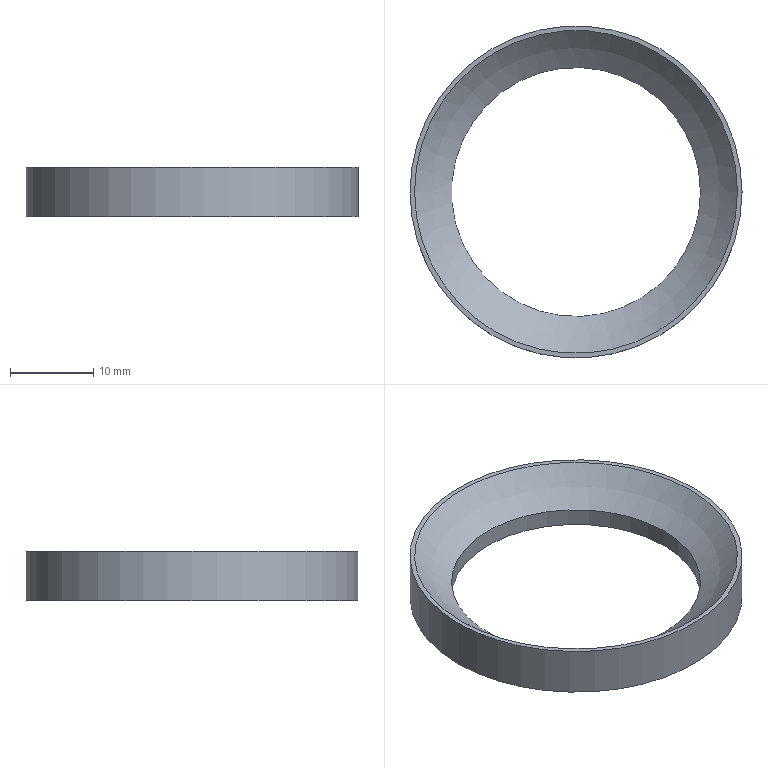Component | NX | CORE_SEAL_2 | 1 solid | 5 faces | box 40 x 40 x 6 mm | volume 2343 mm3 | plane 2 | cylinder 2 | sphere 1 | commonest cylinder face diameters 40 x1 30 x1
STEP:
#1=CARTESIAN_POINT('',(0.,0.,0.));
#2=DIRECTION('',(0.,0.,1.));
#3=DIRECTION('',(1.,0.,0.));
#4=AXIS2_PLACEMENT_3D('',#1,#2,#3);
#5=CARTESIAN_POINT('',(19.449,0.,-45.));
#6=VERTEX_POINT('',#5);
#7=CARTESIAN_POINT('',(0.,0.,-45.));
#8=DIRECTION('',(0.,0.,1.));
#9=DIRECTION('',(1.,0.,0.));
#10=AXIS2_PLACEMENT_3D('',#7,#8,#9);
#11=CIRCLE('',#10,19.449);
#12=CARTESIAN_POINT('',(0.,0.,-45.));
#13=DIRECTION('',(0.,0.,1.));
#14=DIRECTION('',(1.,0.,0.));
#15=AXIS2_PLACEMENT_3D('',#12,#13,#14);
#16=PLANE('',#15);
#17=CARTESIAN_POINT('',(0.,0.));
#18=DIRECTION('',(1.,0.));
#19=AXIS2_PLACEMENT_2D('',#17,#18);
#20=CIRCLE('',#19,19.449);
#21=(GEOMETRIC_REPRESENTATION_CONTEXT(2)PARAMETRIC_REPRESENTATION_CONTEXT()REPRESENTATION_CONTEXT('',''));
#22=DEFINITIONAL_REPRESENTATION('',(#20),#21);
#23=PCURVE('',#16,#22);
#24=CARTESIAN_POINT('',(0.,0.,-27.));
#25=DIRECTION('',(0.,0.,1.));
#26=DIRECTION('',(1.,0.,-0.));
#27=AXIS2_PLACEMENT_3D('',#24,#25,#26);
#28=SPHERICAL_SURFACE('',#27,26.5);
#29=CARTESIAN_POINT('',(0.,-0.7467));
#30=DIRECTION('',(1.,0.));
#31=VECTOR('',#30,1.);
#32=LINE('',#29,#31);
#33=(GEOMETRIC_REPRESENTATION_CONTEXT(2)PARAMETRIC_REPRESENTATION_CONTEXT()REPRESENTATION_CONTEXT('',''));
#34=DEFINITIONAL_REPRESENTATION('',(#32),#33);
#35=PCURVE('',#28,#34);
#36=SURFACE_CURVE('',#11,(#23,#35),.PCURVE_S1.);
#37=EDGE_CURVE('',#6,#6,#36,.T.);
#38=ORIENTED_EDGE('',*,*,#37,.F.);
#39=EDGE_LOOP('',(#38));
#40=FACE_BOUND('',#39,.T.);
#41=CARTESIAN_POINT('',(20.,0.,-45.));
#42=VERTEX_POINT('',#41);
#43=CARTESIAN_POINT('',(0.,0.,-45.));
#44=DIRECTION('',(0.,0.,-1.));
#45=DIRECTION('',(1.,0.,0.));
#46=AXIS2_PLACEMENT_3D('',#43,#44,#45);
#47=CIRCLE('',#46,20.);
#48=CARTESIAN_POINT('',(20.,0.));
#49=CARTESIAN_POINT('',(20.,-34.641));
#50=CARTESIAN_POINT('',(-10.,-17.321));
#51=CARTESIAN_POINT('',(-40.,-0.));
#52=CARTESIAN_POINT('',(-10.,17.321));
#53=CARTESIAN_POINT('',(20.,34.641));
#54=CARTESIAN_POINT('',(20.,0.));
#55=(BOUNDED_CURVE()B_SPLINE_CURVE(2,(#48,#49,#50,#51,#52,#53,#54),.UNSPECIFIED.,.T.,.F.)B_SPLINE_CURVE_WITH_KNOTS((1,2,2,2,2,1),(-2.094,0.,2.094,4.189,6.283,8.378),.UNSPECIFIED.)CURVE()GEOMETRIC_REPRESENTATION_ITEM()RATIONAL_B_SPLINE_CURVE((1.,0.5,1.,0.5,1.,0.5,1.))REPRESENTATION_ITEM(''));
#56=(GEOMETRIC_REPRESENTATION_CONTEXT(2)PARAMETRIC_REPRESENTATION_CONTEXT()REPRESENTATION_CONTEXT('',''));
#57=DEFINITIONAL_REPRESENTATION('',(#55),#56);
#58=PCURVE('',#16,#57);
#59=CARTESIAN_POINT('',(0.,0.,-51.));
#60=DIRECTION('',(0.,0.,1.));
#61=DIRECTION('',(1.,0.,0.));
#62=AXIS2_PLACEMENT_3D('',#59,#60,#61);
#63=CYLINDRICAL_SURFACE('',#62,20.);
#64=CARTESIAN_POINT('',(6.283,6.));
#65=DIRECTION('',(-1.,0.));
#66=VECTOR('',#65,1.);
#67=LINE('',#64,#66);
#68=(GEOMETRIC_REPRESENTATION_CONTEXT(2)PARAMETRIC_REPRESENTATION_CONTEXT()REPRESENTATION_CONTEXT('',''));
#69=DEFINITIONAL_REPRESENTATION('',(#67),#68);
#70=PCURVE('',#63,#69);
#71=SURFACE_CURVE('',#47,(#58,#70),.PCURVE_S1.);
#72=EDGE_CURVE('',#42,#42,#71,.T.);
#73=ORIENTED_EDGE('',*,*,#72,.F.);
#74=EDGE_LOOP('',(#73));
#75=FACE_BOUND('',#74,.T.);
#76=ADVANCED_FACE('',(#40,#75),#16,.T.);
#77=CARTESIAN_POINT('',(15.,0.,-51.));
#78=VERTEX_POINT('',#77);
#79=CARTESIAN_POINT('',(0.,0.,-51.));
#80=DIRECTION('',(0.,0.,1.));
#81=DIRECTION('',(1.,0.,0.));
#82=AXIS2_PLACEMENT_3D('',#79,#80,#81);
#83=CIRCLE('',#82,15.);
#84=CARTESIAN_POINT('',(0.,0.,-51.));
#85=DIRECTION('',(0.,0.,-1.));
#86=DIRECTION('',(-1.,0.,0.));
#87=AXIS2_PLACEMENT_3D('',#84,#85,#86);
#88=PLANE('',#87);
#89=CARTESIAN_POINT('',(-15.,0.));
#90=CARTESIAN_POINT('',(-15.,25.981));
#91=CARTESIAN_POINT('',(7.5,12.99));
#92=CARTESIAN_POINT('',(30.,0.));
#93=CARTESIAN_POINT('',(7.5,-12.99));
#94=CARTESIAN_POINT('',(-15.,-25.981));
#95=CARTESIAN_POINT('',(-15.,0.));
#96=(BOUNDED_CURVE()B_SPLINE_CURVE(2,(#89,#90,#91,#92,#93,#94,#95),.UNSPECIFIED.,.T.,.F.)B_SPLINE_CURVE_WITH_KNOTS((1,2,2,2,2,1),(-2.094,0.,2.094,4.189,6.283,8.378),.UNSPECIFIED.)CURVE()GEOMETRIC_REPRESENTATION_ITEM()RATIONAL_B_SPLINE_CURVE((1.,0.5,1.,0.5,1.,0.5,1.))REPRESENTATION_ITEM(''));
#97=(GEOMETRIC_REPRESENTATION_CONTEXT(2)PARAMETRIC_REPRESENTATION_CONTEXT()REPRESENTATION_CONTEXT('',''));
#98=DEFINITIONAL_REPRESENTATION('',(#96),#97);
#99=PCURVE('',#88,#98);
#100=CARTESIAN_POINT('',(0.,0.,-51.));
#101=DIRECTION('',(0.,0.,1.));
#102=DIRECTION('',(1.,0.,0.));
#103=AXIS2_PLACEMENT_3D('',#100,#101,#102);
#104=CYLINDRICAL_SURFACE('',#103,15.);
#105=CARTESIAN_POINT('',(0.,0.));
#106=DIRECTION('',(1.,0.));
#107=VECTOR('',#106,1.);
#108=LINE('',#105,#107);
#109=(GEOMETRIC_REPRESENTATION_CONTEXT(2)PARAMETRIC_REPRESENTATION_CONTEXT()REPRESENTATION_CONTEXT('',''));
#110=DEFINITIONAL_REPRESENTATION('',(#108),#109);
#111=PCURVE('',#104,#110);
#112=SURFACE_CURVE('',#83,(#99,#111),.PCURVE_S1.);
#113=EDGE_CURVE('',#78,#78,#112,.T.);
#114=ORIENTED_EDGE('',*,*,#113,.T.);
#115=EDGE_LOOP('',(#114));
#116=FACE_BOUND('',#115,.T.);
#117=CARTESIAN_POINT('',(20.,0.,-51.));
#118=VERTEX_POINT('',#117);
#119=CARTESIAN_POINT('',(0.,0.,-51.));
#120=DIRECTION('',(0.,0.,1.));
#121=DIRECTION('',(1.,0.,0.));
#122=AXIS2_PLACEMENT_3D('',#119,#120,#121);
#123=CIRCLE('',#122,20.);
#124=CARTESIAN_POINT('',(-20.,0.));
#125=CARTESIAN_POINT('',(-20.,34.641));
#126=CARTESIAN_POINT('',(10.,17.321));
#127=CARTESIAN_POINT('',(40.,0.));
#128=CARTESIAN_POINT('',(10.,-17.321));
#129=CARTESIAN_POINT('',(-20.,-34.641));
#130=CARTESIAN_POINT('',(-20.,0.));
#131=(BOUNDED_CURVE()B_SPLINE_CURVE(2,(#124,#125,#126,#127,#128,#129,#130),.UNSPECIFIED.,.T.,.F.)B_SPLINE_CURVE_WITH_KNOTS((1,2,2,2,2,1),(-2.094,0.,2.094,4.189,6.283,8.378),.UNSPECIFIED.)CURVE()GEOMETRIC_REPRESENTATION_ITEM()RATIONAL_B_SPLINE_CURVE((1.,0.5,1.,0.5,1.,0.5,1.))REPRESENTATION_ITEM(''));
#132=(GEOMETRIC_REPRESENTATION_CONTEXT(2)PARAMETRIC_REPRESENTATION_CONTEXT()REPRESENTATION_CONTEXT('',''));
#133=DEFINITIONAL_REPRESENTATION('',(#131),#132);
#134=PCURVE('',#88,#133);
#135=CARTESIAN_POINT('',(0.,0.));
#136=DIRECTION('',(1.,0.));
#137=VECTOR('',#136,1.);
#138=LINE('',#135,#137);
#139=(GEOMETRIC_REPRESENTATION_CONTEXT(2)PARAMETRIC_REPRESENTATION_CONTEXT()REPRESENTATION_CONTEXT('',''));
#140=DEFINITIONAL_REPRESENTATION('',(#138),#139);
#141=PCURVE('',#63,#140);
#142=SURFACE_CURVE('',#123,(#134,#141),.PCURVE_S1.);
#143=EDGE_CURVE('',#118,#118,#142,.T.);
#144=ORIENTED_EDGE('',*,*,#143,.F.);
#145=EDGE_LOOP('',(#144));
#146=FACE_BOUND('',#145,.T.);
#147=ADVANCED_FACE('',(#116,#146),#88,.T.);
#148=ORIENTED_EDGE('',*,*,#72,.T.);
#149=CARTESIAN_POINT('',(20.,-0.,-51.));
#150=CARTESIAN_POINT('',(20.,-0.,-45.));
#151=B_SPLINE_CURVE_WITH_KNOTS('',1,(#149,#150),.UNSPECIFIED.,.F.,.F.,(2,2),(0.,6.),.PIECEWISE_BEZIER_KNOTS.);
#152=CARTESIAN_POINT('',(0.,0.));
#153=DIRECTION('',(0.,1.));
#154=VECTOR('',#153,1.);
#155=LINE('',#152,#154);
#156=(GEOMETRIC_REPRESENTATION_CONTEXT(2)PARAMETRIC_REPRESENTATION_CONTEXT()REPRESENTATION_CONTEXT('',''));
#157=DEFINITIONAL_REPRESENTATION('',(#155),#156);
#158=PCURVE('',#63,#157);
#159=CARTESIAN_POINT('',(6.283,0.));
#160=DIRECTION('',(0.,1.));
#161=VECTOR('',#160,1.);
#162=LINE('',#159,#161);
#163=(GEOMETRIC_REPRESENTATION_CONTEXT(2)PARAMETRIC_REPRESENTATION_CONTEXT()REPRESENTATION_CONTEXT('',''));
#164=DEFINITIONAL_REPRESENTATION('',(#162),#163);
#165=PCURVE('',#63,#164);
#166=SEAM_CURVE('',#151,(#158,#165),.PCURVE_S1.);
#167=EDGE_CURVE('',#118,#42,#166,.T.);
#168=ORIENTED_EDGE('',*,*,#167,.F.);
#169=ORIENTED_EDGE('',*,*,#143,.T.);
#170=ORIENTED_EDGE('',*,*,#167,.T.);
#171=EDGE_LOOP('',(#148,#168,#169,#170));
#172=FACE_BOUND('',#171,.T.);
#173=ADVANCED_FACE('',(#172),#63,.T.);
#174=CARTESIAN_POINT('',(15.,0.,-48.846));
#175=VERTEX_POINT('',#174);
#176=CARTESIAN_POINT('',(0.,0.,-48.846));
#177=DIRECTION('',(0.,0.,-1.));
#178=DIRECTION('',(1.,0.,0.));
#179=AXIS2_PLACEMENT_3D('',#176,#177,#178);
#180=CIRCLE('',#179,15.);
#181=CARTESIAN_POINT('',(6.283,-0.9691));
#182=CARTESIAN_POINT('',(6.188,-0.9691));
#183=CARTESIAN_POINT('',(5.998,-0.9691));
#184=CARTESIAN_POINT('',(5.712,-0.9691));
#185=CARTESIAN_POINT('',(5.426,-0.9691));
#186=CARTESIAN_POINT('',(5.141,-0.9691));
#187=CARTESIAN_POINT('',(4.855,-0.9691));
#188=CARTESIAN_POINT('',(4.57,-0.9691));
#189=CARTESIAN_POINT('',(4.284,-0.9691));
#190=CARTESIAN_POINT('',(3.998,-0.9691));
#191=CARTESIAN_POINT('',(3.713,-0.9691));
#192=CARTESIAN_POINT('',(3.427,-0.9691));
#193=CARTESIAN_POINT('',(3.142,-0.9691));
#194=CARTESIAN_POINT('',(2.856,-0.9691));
#195=CARTESIAN_POINT('',(2.57,-0.9691));
#196=CARTESIAN_POINT('',(2.285,-0.9691));
#197=CARTESIAN_POINT('',(1.999,-0.9691));
#198=CARTESIAN_POINT('',(1.714,-0.9691));
#199=CARTESIAN_POINT('',(1.428,-0.9691));
#200=CARTESIAN_POINT('',(1.142,-0.9691));
#201=CARTESIAN_POINT('',(0.8568,-0.9691));
#202=CARTESIAN_POINT('',(0.5712,-0.9691));
#203=CARTESIAN_POINT('',(0.2856,-0.9691));
#204=CARTESIAN_POINT('',(0.0952,-0.9691));
#205=CARTESIAN_POINT('',(0.,-0.9691));
#206=B_SPLINE_CURVE_WITH_KNOTS('',3,(#181,#182,#183,#184,#185,#186,#187,#188,#189,#190,#191,#192,#193,#194,#195,#196,#197,#198,#199,#200,#201,#202,#203,#204,#205),.UNSPECIFIED.,.F.,.F.,(4,1,1,1,1,1,1,1,1,1,1,1,1,1,1,1,1,1,1,1,1,1,4),(0.,0.2856,0.5712,0.8568,1.142,1.428,1.714,1.999,2.285,2.57,2.856,3.142,3.427,3.713,3.998,4.284,4.57,4.855,5.141,5.426,5.712,5.998,6.283),.QUASI_UNIFORM_KNOTS.);
#207=(GEOMETRIC_REPRESENTATION_CONTEXT(2)PARAMETRIC_REPRESENTATION_CONTEXT()REPRESENTATION_CONTEXT('',''));
#208=DEFINITIONAL_REPRESENTATION('',(#206),#207);
#209=PCURVE('',#28,#208);
#210=CARTESIAN_POINT('',(6.283,2.154));
#211=DIRECTION('',(-1.,0.));
#212=VECTOR('',#211,1.);
#213=LINE('',#210,#212);
#214=(GEOMETRIC_REPRESENTATION_CONTEXT(2)PARAMETRIC_REPRESENTATION_CONTEXT()REPRESENTATION_CONTEXT('',''));
#215=DEFINITIONAL_REPRESENTATION('',(#213),#214);
#216=PCURVE('',#104,#215);
#217=SURFACE_CURVE('',#180,(#209,#216),.PCURVE_S1.);
#218=EDGE_CURVE('',#175,#175,#217,.T.);
#219=ORIENTED_EDGE('',*,*,#218,.F.);
#220=CARTESIAN_POINT('',(15.,0.,-48.846));
#221=CARTESIAN_POINT('',(16.214,0.,-48.012));
#222=CARTESIAN_POINT('',(17.367,0.,-47.088));
#223=CARTESIAN_POINT('',(18.448,0.,-46.081));
#224=CARTESIAN_POINT('',(19.449,0.,-45.));
#225=B_SPLINE_CURVE_WITH_KNOTS('',4,(#220,#221,#222,#223,#224),.UNSPECIFIED.,.F.,.F.,(5,5),(-0.9691,-0.7467),.PIECEWISE_BEZIER_KNOTS.);
#226=CARTESIAN_POINT('',(6.283,0.));
#227=DIRECTION('',(0.,1.));
#228=VECTOR('',#227,1.);
#229=LINE('',#226,#228);
#230=(GEOMETRIC_REPRESENTATION_CONTEXT(2)PARAMETRIC_REPRESENTATION_CONTEXT()REPRESENTATION_CONTEXT('',''));
#231=DEFINITIONAL_REPRESENTATION('',(#229),#230);
#232=PCURVE('',#28,#231);
#233=CARTESIAN_POINT('',(0.,0.));
#234=DIRECTION('',(0.,1.));
#235=VECTOR('',#234,1.);
#236=LINE('',#233,#235);
#237=(GEOMETRIC_REPRESENTATION_CONTEXT(2)PARAMETRIC_REPRESENTATION_CONTEXT()REPRESENTATION_CONTEXT('',''));
#238=DEFINITIONAL_REPRESENTATION('',(#236),#237);
#239=PCURVE('',#28,#238);
#240=SEAM_CURVE('',#225,(#232,#239),.PCURVE_S1.);
#241=EDGE_CURVE('',#175,#6,#240,.T.);
#242=ORIENTED_EDGE('',*,*,#241,.T.);
#243=ORIENTED_EDGE('',*,*,#37,.F.);
#244=ORIENTED_EDGE('',*,*,#241,.F.);
#245=EDGE_LOOP('',(#219,#242,#243,#244));
#246=FACE_BOUND('',#245,.F.);
#247=ADVANCED_FACE('',(#246),#28,.F.);
#248=ORIENTED_EDGE('',*,*,#113,.T.);
#249=CARTESIAN_POINT('',(15.,0.,-51.));
#250=CARTESIAN_POINT('',(15.,0.,-48.846));
#251=B_SPLINE_CURVE_WITH_KNOTS('',1,(#249,#250),.UNSPECIFIED.,.F.,.F.,(2,2),(0.,2.154),.PIECEWISE_BEZIER_KNOTS.);
#252=CARTESIAN_POINT('',(6.283,0.));
#253=DIRECTION('',(0.,1.));
#254=VECTOR('',#253,1.);
#255=LINE('',#252,#254);
#256=(GEOMETRIC_REPRESENTATION_CONTEXT(2)PARAMETRIC_REPRESENTATION_CONTEXT()REPRESENTATION_CONTEXT('',''));
#257=DEFINITIONAL_REPRESENTATION('',(#255),#256);
#258=PCURVE('',#104,#257);
#259=CARTESIAN_POINT('',(0.,0.));
#260=DIRECTION('',(0.,1.));
#261=VECTOR('',#260,1.);
#262=LINE('',#259,#261);
#263=(GEOMETRIC_REPRESENTATION_CONTEXT(2)PARAMETRIC_REPRESENTATION_CONTEXT()REPRESENTATION_CONTEXT('',''));
#264=DEFINITIONAL_REPRESENTATION('',(#262),#263);
#265=PCURVE('',#104,#264);
#266=SEAM_CURVE('',#251,(#258,#265),.PCURVE_S1.);
#267=EDGE_CURVE('',#78,#175,#266,.T.);
#268=ORIENTED_EDGE('',*,*,#267,.T.);
#269=ORIENTED_EDGE('',*,*,#218,.T.);
#270=ORIENTED_EDGE('',*,*,#267,.F.);
#271=EDGE_LOOP('',(#248,#268,#269,#270));
#272=FACE_BOUND('',#271,.F.);
#273=ADVANCED_FACE('',(#272),#104,.F.);
#274=CLOSED_SHELL('',(#76,#147,#173,#247,#273));
#275=MANIFOLD_SOLID_BREP('',#274);
#276=(LENGTH_UNIT()NAMED_UNIT(*)SI_UNIT(.MILLI.,.METRE.));
#277=UNCERTAINTY_MEASURE_WITH_UNIT(LENGTH_MEASURE(0.00001),#276,'','');
#278=(NAMED_UNIT(*)PLANE_ANGLE_UNIT()SI_UNIT($,.RADIAN.));
#279=(NAMED_UNIT(*)SI_UNIT($,.STERADIAN.)SOLID_ANGLE_UNIT());
#280=(GEOMETRIC_REPRESENTATION_CONTEXT(3)GLOBAL_UNCERTAINTY_ASSIGNED_CONTEXT((#277))GLOBAL_UNIT_ASSIGNED_CONTEXT((#276,#278,#279))REPRESENTATION_CONTEXT('',''));
#281=ADVANCED_BREP_SHAPE_REPRESENTATION('',(#4,#275),#280);